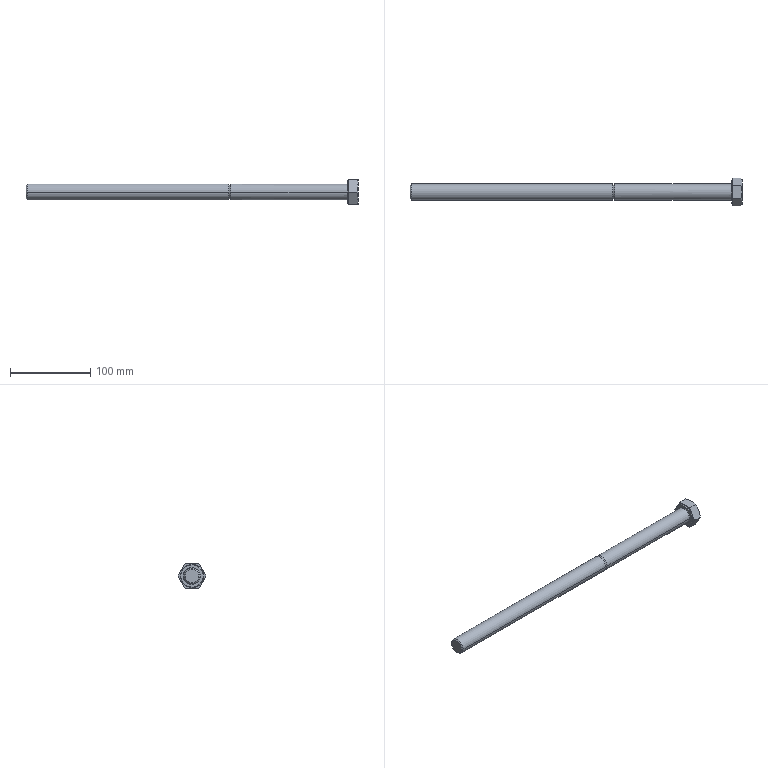Component | NX | BOLT_M20X400 | 1 solid | 31 faces | volume 135107 mm3 | cone 12 | plane 11 | cylinder 4 | torus 4 | commonest cylinder face diameters 20 x4